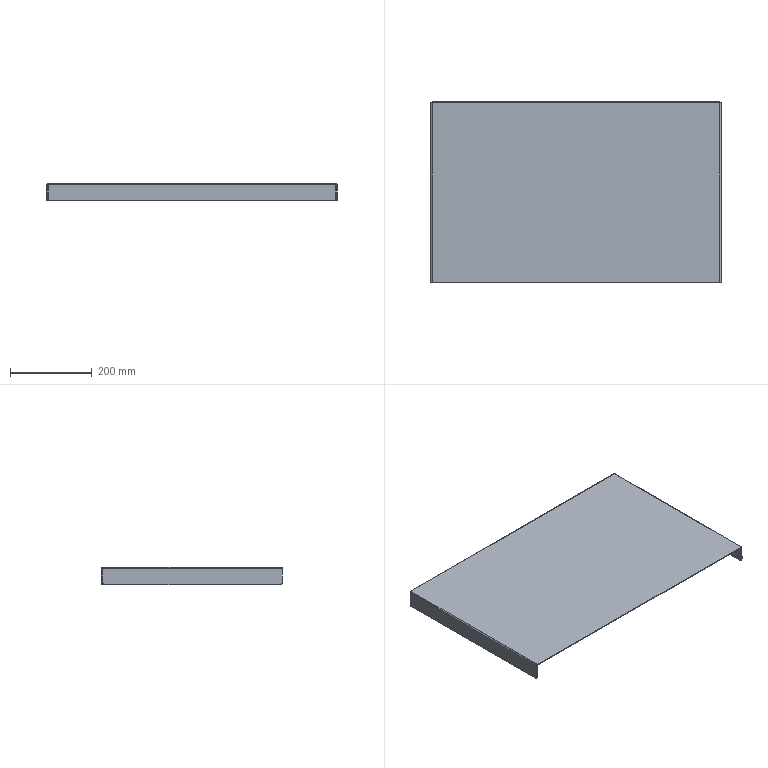Component | SolidWorks | HFS8_4545_09-B-2 | 1 solid | 36 faces | volume 751840 mm3 | plane 20 | cylinder 12 | spline 4 | commonest cylinder face diameters 10 x6 5.473 x3 1.473 x3 | material Stainless Steel (Ferritic)